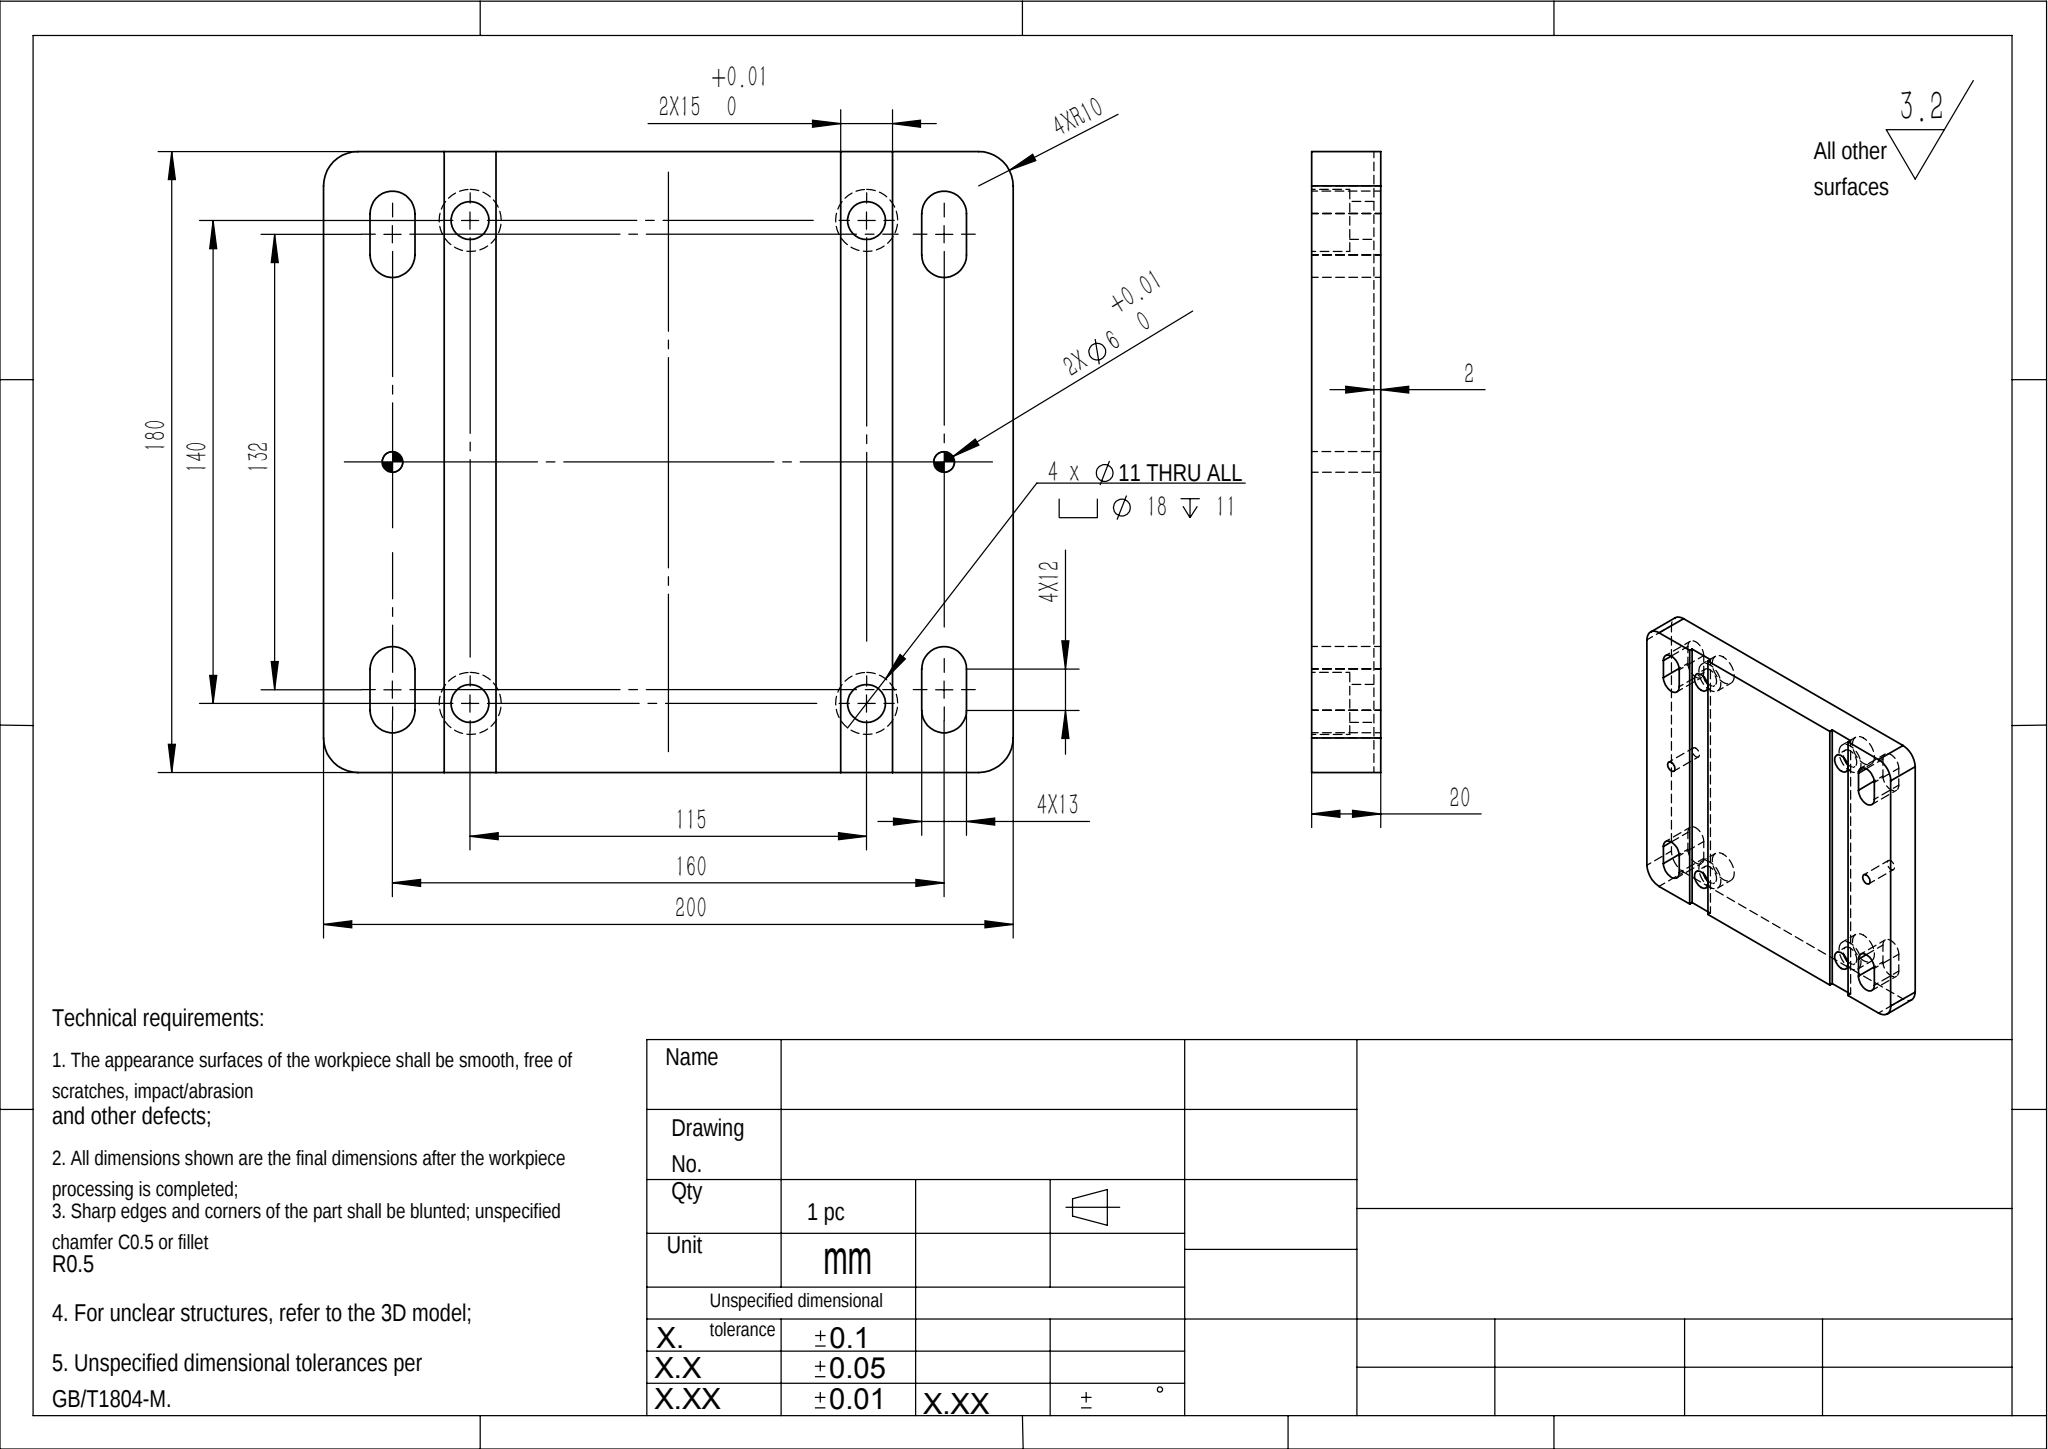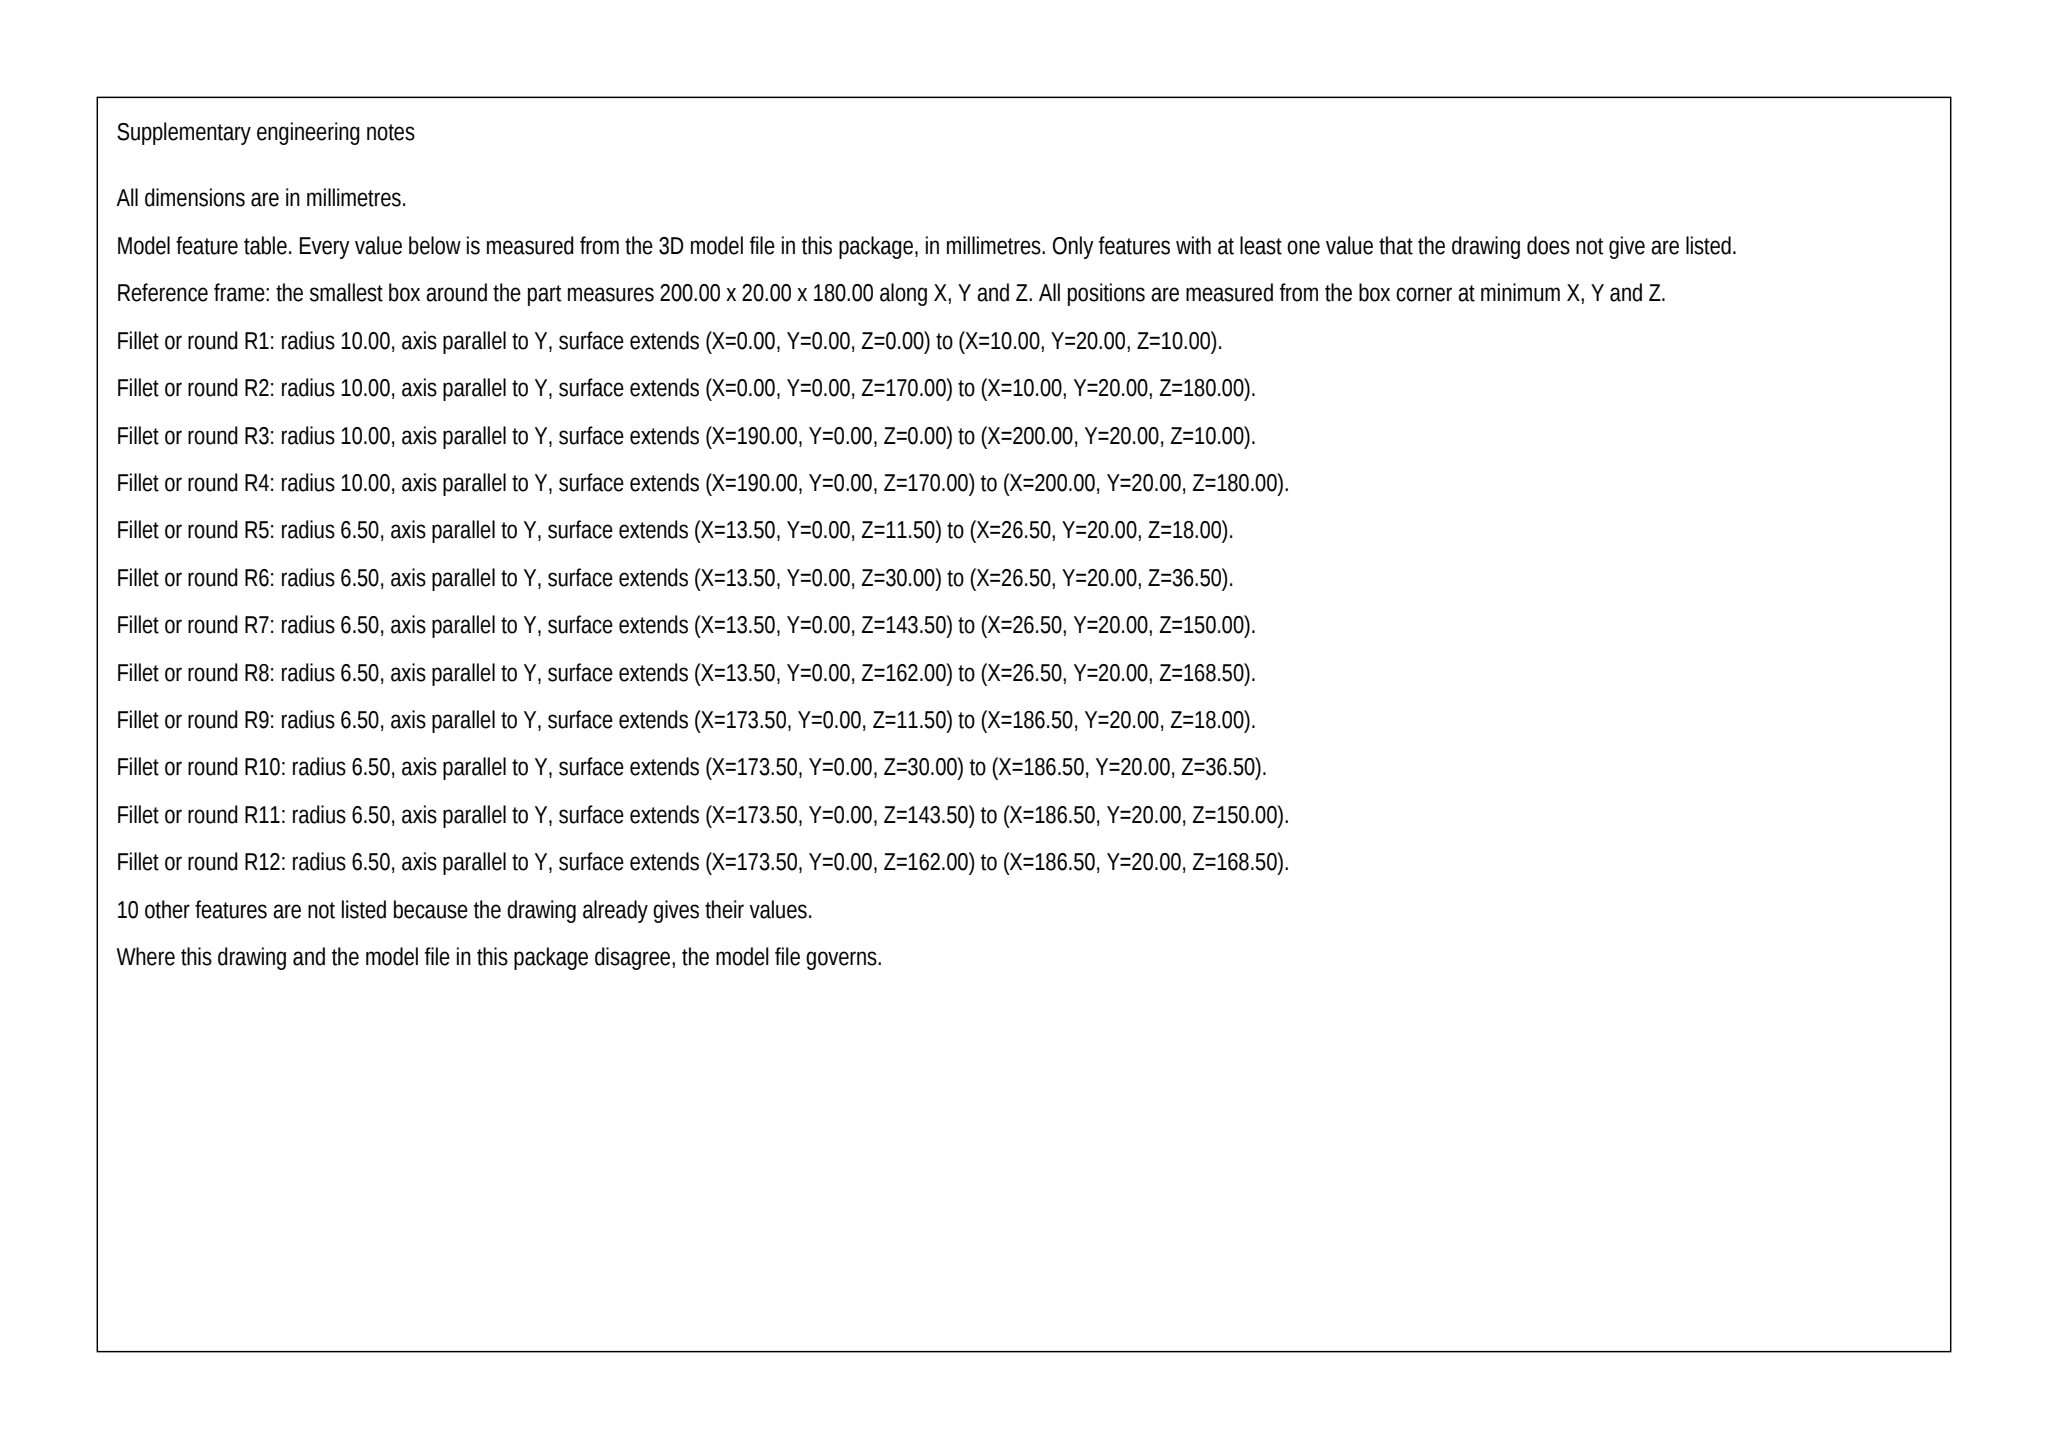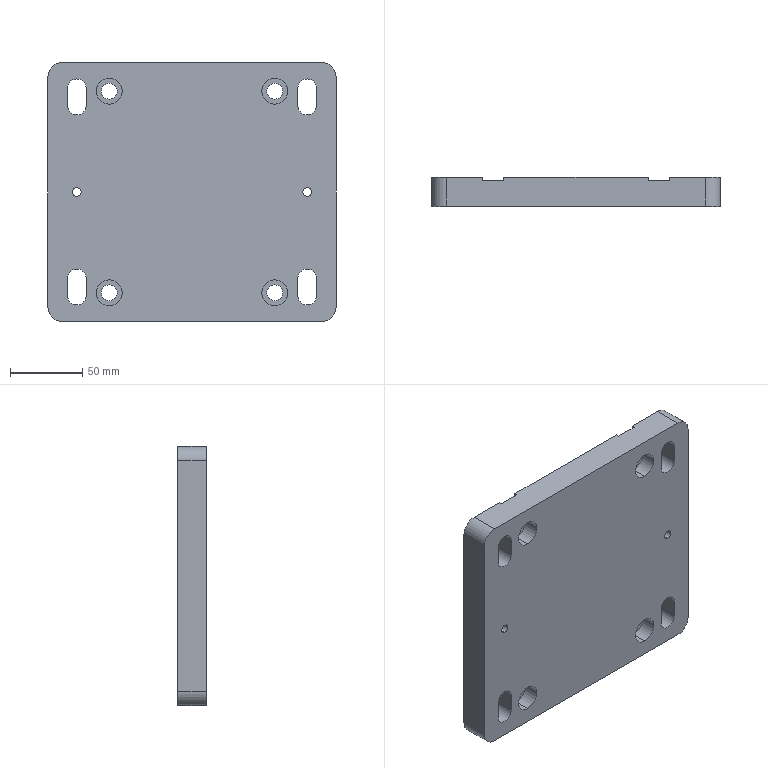Part | SolidWorks | mm | 1 solid | 62 faces | box 200 x 20 x 180 mm | volume 669396 mm3 | cylinder 36 | plane 26 | commonest cylinder face diameters 13 x12 18 x8 11 x8 6 x4 20 x4
build123d program:
from build123d import *

# Parameters (mm, degrees)
SKETCH1_W                                         = 200
SKETCH1_H                                         = 180
BOSS_EXTRUDE1_DEPTH                               = 20
FILLET1_R                                         = 10
SKETCH10_W                                        = 15
SKETCH10_H                                        = 180
CUT_EXTRUDE4_DEPTH                                = 2
HOLE_SIZE_ACCORDING_TO_HEXAGON_SOCKET_D           = 11
HOLE_SIZE_ACCORDING_TO_HEXAGON_SOCKET_CBORE_D     = 18
HOLE_SIZE_ACCORDING_TO_HEXAGON_SOCKET_CBORE_DEPTH = 11
CUT_EXTRUDE5_DEPTH                                = 137.015
SIZE_MM_DOWEL_PIN_HOLE_1_D                        = 6


with BuildPart() as part:
    # Sketch1 → Boss-Extrude1 (new body)
    with BuildSketch(Plane(origin=(0, 0, 0), x_dir=(1, 0, 0), z_dir=(0, 1, 0))):
        Rectangle(SKETCH1_W, SKETCH1_H)
    extrude(amount=BOSS_EXTRUDE1_DEPTH)

    # Fillet1
    fillet1_edges = [part.edges().sort_by_distance(p)[0] for p in [
        (100, 10, -90),
        (100, 10, 90),
        (-100, 10, 90),
        (-100, 10, -90),
    ]]
    fillet(fillet1_edges, radius=FILLET1_R)

    # Sketch10 → Cut-Extrude4 (cut)
    with BuildSketch(Plane(origin=(0, 20, 0), x_dir=(1, 0, 0), z_dir=(0, 1, 0))):
        with Locations((-57.5, 0)):
            Rectangle(SKETCH10_W, SKETCH10_H)
        with Locations((57.5, 0)):
            Rectangle(SKETCH10_W, SKETCH10_H)
    extrude(amount=-CUT_EXTRUDE4_DEPTH, mode=Mode.SUBTRACT)

    # Hole Size _ according to_ Hexagon Socket (through all)
    with Locations(Plane(origin=(-57.5, 0, 70), x_dir=(0, 0, -1), z_dir=(0, -1, 0))):
        with Locations((0, 0), (140, 0), (140, 115), (0, 115)):
            CounterBoreHole(HOLE_SIZE_ACCORDING_TO_HEXAGON_SOCKET_D / 2, HOLE_SIZE_ACCORDING_TO_HEXAGON_SOCKET_CBORE_D / 2, HOLE_SIZE_ACCORDING_TO_HEXAGON_SOCKET_CBORE_DEPTH)

    # Sketch13 → Cut-Extrude5 (cut, through all)
    with BuildSketch(Plane(origin=(0, 20, 0), x_dir=(1, 0, 0), z_dir=(0, 1, 0))):
        with BuildLine():
            Line((-86.5, 60), (-86.5, 72))
            ThreePointArc((-86.5, 72), (-80, 78.5), (-73.5, 72))
            Line((-73.5, 72), (-73.5, 60))
            ThreePointArc((-73.5, 60), (-80, 53.5), (-86.5, 60))
        make_face()
        with BuildLine():
            Line((73.5, 60), (73.5, 72))
            ThreePointArc((73.5, 72), (80, 78.5), (86.5, 72))
            Line((86.5, 72), (86.5, 60))
            ThreePointArc((86.5, 60), (80, 53.5), (73.5, 60))
        make_face()
        with BuildLine():
            Line((86.5, -60), (86.5, -72))
            ThreePointArc((86.5, -72), (80, -78.5), (73.5, -72))
            Line((73.5, -72), (73.5, -60))
            ThreePointArc((73.5, -60), (80, -53.5), (86.5, -60))
        make_face()
        with BuildLine():
            Line((-73.5, -60), (-73.5, -72))
            ThreePointArc((-73.5, -72), (-80, -78.5), (-86.5, -72))
            Line((-86.5, -72), (-86.5, -60))
            ThreePointArc((-86.5, -60), (-80, -53.5), (-73.5, -60))
        make_face()
    extrude(amount=-CUT_EXTRUDE5_DEPTH, mode=Mode.SUBTRACT)

    # Size mm Dowel Pin Hole 1 (through all)
    with Locations(Plane(origin=(-80, 0, 0), x_dir=(0, 0, -1), z_dir=(0, -1, 0))):
        with Locations((0, 0), (0, 160)):
            Hole(SIZE_MM_DOWEL_PIN_HOLE_1_D / 2)


solid = part.part